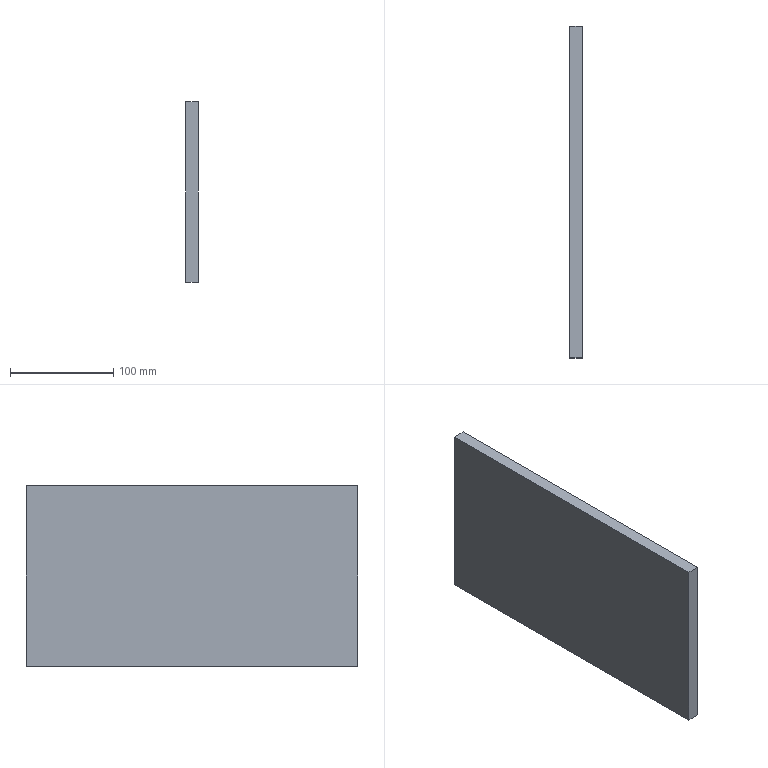Component | NX | CH3404_5-12 | 1 solid | 6 faces | box 12 x 321 x 175 mm | volume 674100 mm3 | plane 6
STEP:
#1=CARTESIAN_POINT('',(0.,0.,0.));
#2=DIRECTION('',(0.,0.,1.));
#3=DIRECTION('',(1.,0.,0.));
#4=AXIS2_PLACEMENT_3D('',#1,#2,#3);
#5=CARTESIAN_POINT('',(-155.,-160.5,1775.));
#6=VERTEX_POINT('',#5);
#7=CARTESIAN_POINT('',(-155.,-160.5,1600.));
#8=VERTEX_POINT('',#7);
#9=CARTESIAN_POINT('',(-155.,-160.5,1775.));
#10=DIRECTION('',(0.,0.,-1.));
#11=VECTOR('',#10,1.);
#12=LINE('',#9,#11);
#13=CARTESIAN_POINT('',(-143.,-160.5,1775.));
#14=DIRECTION('',(0.,1.,0.));
#15=DIRECTION('',(0.,0.,1.));
#16=AXIS2_PLACEMENT_3D('',#13,#14,#15);
#17=PLANE('',#16);
#18=CARTESIAN_POINT('',(0.,-12.));
#19=DIRECTION('',(-1.,0.));
#20=VECTOR('',#19,1.);
#21=LINE('',#18,#20);
#22=(GEOMETRIC_REPRESENTATION_CONTEXT(2)PARAMETRIC_REPRESENTATION_CONTEXT()REPRESENTATION_CONTEXT('',''));
#23=DEFINITIONAL_REPRESENTATION('',(#21),#22);
#24=PCURVE('',#17,#23);
#25=CARTESIAN_POINT('',(-155.,0.,1687.5));
#26=DIRECTION('',(1.,0.,0.));
#27=DIRECTION('',(0.,0.,-1.));
#28=AXIS2_PLACEMENT_3D('',#25,#26,#27);
#29=PLANE('',#28);
#30=CARTESIAN_POINT('',(-87.5,-160.5));
#31=DIRECTION('',(1.,0.));
#32=VECTOR('',#31,1.);
#33=LINE('',#30,#32);
#34=(GEOMETRIC_REPRESENTATION_CONTEXT(2)PARAMETRIC_REPRESENTATION_CONTEXT()REPRESENTATION_CONTEXT('',''));
#35=DEFINITIONAL_REPRESENTATION('',(#33),#34);
#36=PCURVE('',#29,#35);
#37=SURFACE_CURVE('',#12,(#24,#36),.PCURVE_S1.);
#38=EDGE_CURVE('',#6,#8,#37,.T.);
#39=ORIENTED_EDGE('',*,*,#38,.T.);
#40=CARTESIAN_POINT('',(-143.,-160.5,1600.));
#41=VERTEX_POINT('',#40);
#42=CARTESIAN_POINT('',(-143.,-160.5,1600.));
#43=DIRECTION('',(-1.,0.,0.));
#44=VECTOR('',#43,1.);
#45=LINE('',#42,#44);
#46=CARTESIAN_POINT('',(-175.,0.));
#47=DIRECTION('',(0.,-1.));
#48=VECTOR('',#47,1.);
#49=LINE('',#46,#48);
#50=(GEOMETRIC_REPRESENTATION_CONTEXT(2)PARAMETRIC_REPRESENTATION_CONTEXT()REPRESENTATION_CONTEXT('',''));
#51=DEFINITIONAL_REPRESENTATION('',(#49),#50);
#52=PCURVE('',#17,#51);
#53=CARTESIAN_POINT('',(-143.,-160.5,1600.));
#54=DIRECTION('',(0.,0.,1.));
#55=DIRECTION('',(1.,0.,0.));
#56=AXIS2_PLACEMENT_3D('',#53,#54,#55);
#57=PLANE('',#56);
#58=CARTESIAN_POINT('',(0.,0.));
#59=DIRECTION('',(-1.,0.));
#60=VECTOR('',#59,1.);
#61=LINE('',#58,#60);
#62=(GEOMETRIC_REPRESENTATION_CONTEXT(2)PARAMETRIC_REPRESENTATION_CONTEXT()REPRESENTATION_CONTEXT('',''));
#63=DEFINITIONAL_REPRESENTATION('',(#61),#62);
#64=PCURVE('',#57,#63);
#65=SURFACE_CURVE('',#45,(#52,#64),.PCURVE_S1.);
#66=EDGE_CURVE('',#41,#8,#65,.T.);
#67=ORIENTED_EDGE('',*,*,#66,.F.);
#68=CARTESIAN_POINT('',(-143.,-160.5,1775.));
#69=VERTEX_POINT('',#68);
#70=CARTESIAN_POINT('',(-143.,-160.5,1775.));
#71=DIRECTION('',(0.,0.,-1.));
#72=VECTOR('',#71,1.);
#73=LINE('',#70,#72);
#74=CARTESIAN_POINT('',(0.,0.));
#75=DIRECTION('',(-1.,0.));
#76=VECTOR('',#75,1.);
#77=LINE('',#74,#76);
#78=(GEOMETRIC_REPRESENTATION_CONTEXT(2)PARAMETRIC_REPRESENTATION_CONTEXT()REPRESENTATION_CONTEXT('',''));
#79=DEFINITIONAL_REPRESENTATION('',(#77),#78);
#80=PCURVE('',#17,#79);
#81=CARTESIAN_POINT('',(-143.,0.,1687.5));
#82=DIRECTION('',(1.,0.,0.));
#83=DIRECTION('',(0.,0.,-1.));
#84=AXIS2_PLACEMENT_3D('',#81,#82,#83);
#85=PLANE('',#84);
#86=CARTESIAN_POINT('',(-87.5,-160.5));
#87=DIRECTION('',(1.,0.));
#88=VECTOR('',#87,1.);
#89=LINE('',#86,#88);
#90=(GEOMETRIC_REPRESENTATION_CONTEXT(2)PARAMETRIC_REPRESENTATION_CONTEXT()REPRESENTATION_CONTEXT('',''));
#91=DEFINITIONAL_REPRESENTATION('',(#89),#90);
#92=PCURVE('',#85,#91);
#93=SURFACE_CURVE('',#73,(#80,#92),.PCURVE_S1.);
#94=EDGE_CURVE('',#69,#41,#93,.T.);
#95=ORIENTED_EDGE('',*,*,#94,.F.);
#96=CARTESIAN_POINT('',(-143.,-160.5,1775.));
#97=DIRECTION('',(-1.,0.,0.));
#98=VECTOR('',#97,1.);
#99=LINE('',#96,#98);
#100=CARTESIAN_POINT('',(0.,0.));
#101=DIRECTION('',(0.,-1.));
#102=VECTOR('',#101,1.);
#103=LINE('',#100,#102);
#104=(GEOMETRIC_REPRESENTATION_CONTEXT(2)PARAMETRIC_REPRESENTATION_CONTEXT()REPRESENTATION_CONTEXT('',''));
#105=DEFINITIONAL_REPRESENTATION('',(#103),#104);
#106=PCURVE('',#17,#105);
#107=CARTESIAN_POINT('',(-143.,160.5,1775.));
#108=DIRECTION('',(0.,0.,-1.));
#109=DIRECTION('',(-1.,0.,0.));
#110=AXIS2_PLACEMENT_3D('',#107,#108,#109);
#111=PLANE('',#110);
#112=CARTESIAN_POINT('',(0.,-321.));
#113=DIRECTION('',(1.,0.));
#114=VECTOR('',#113,1.);
#115=LINE('',#112,#114);
#116=(GEOMETRIC_REPRESENTATION_CONTEXT(2)PARAMETRIC_REPRESENTATION_CONTEXT()REPRESENTATION_CONTEXT('',''));
#117=DEFINITIONAL_REPRESENTATION('',(#115),#116);
#118=PCURVE('',#111,#117);
#119=SURFACE_CURVE('',#99,(#106,#118),.PCURVE_S1.);
#120=EDGE_CURVE('',#69,#6,#119,.T.);
#121=ORIENTED_EDGE('',*,*,#120,.T.);
#122=EDGE_LOOP('',(#39,#67,#95,#121));
#123=FACE_BOUND('',#122,.T.);
#124=ADVANCED_FACE('',(#123),#17,.F.);
#125=CARTESIAN_POINT('',(-155.,160.5,1600.));
#126=VERTEX_POINT('',#125);
#127=CARTESIAN_POINT('',(-155.,-160.5,1600.));
#128=DIRECTION('',(0.,1.,0.));
#129=VECTOR('',#128,1.);
#130=LINE('',#127,#129);
#131=CARTESIAN_POINT('',(-12.,0.));
#132=DIRECTION('',(0.,1.));
#133=VECTOR('',#132,1.);
#134=LINE('',#131,#133);
#135=(GEOMETRIC_REPRESENTATION_CONTEXT(2)PARAMETRIC_REPRESENTATION_CONTEXT()REPRESENTATION_CONTEXT('',''));
#136=DEFINITIONAL_REPRESENTATION('',(#134),#135);
#137=PCURVE('',#57,#136);
#138=CARTESIAN_POINT('',(87.5,-160.5));
#139=DIRECTION('',(0.,1.));
#140=VECTOR('',#139,1.);
#141=LINE('',#138,#140);
#142=(GEOMETRIC_REPRESENTATION_CONTEXT(2)PARAMETRIC_REPRESENTATION_CONTEXT()REPRESENTATION_CONTEXT('',''));
#143=DEFINITIONAL_REPRESENTATION('',(#141),#142);
#144=PCURVE('',#29,#143);
#145=SURFACE_CURVE('',#130,(#137,#144),.PCURVE_S1.);
#146=EDGE_CURVE('',#8,#126,#145,.T.);
#147=ORIENTED_EDGE('',*,*,#146,.T.);
#148=CARTESIAN_POINT('',(-143.,160.5,1600.));
#149=VERTEX_POINT('',#148);
#150=CARTESIAN_POINT('',(-143.,160.5,1600.));
#151=DIRECTION('',(-1.,0.,0.));
#152=VECTOR('',#151,1.);
#153=LINE('',#150,#152);
#154=CARTESIAN_POINT('',(0.,321.));
#155=DIRECTION('',(-1.,0.));
#156=VECTOR('',#155,1.);
#157=LINE('',#154,#156);
#158=(GEOMETRIC_REPRESENTATION_CONTEXT(2)PARAMETRIC_REPRESENTATION_CONTEXT()REPRESENTATION_CONTEXT('',''));
#159=DEFINITIONAL_REPRESENTATION('',(#157),#158);
#160=PCURVE('',#57,#159);
#161=CARTESIAN_POINT('',(-143.,160.5,1600.));
#162=DIRECTION('',(0.,-1.,0.));
#163=DIRECTION('',(0.,0.,-1.));
#164=AXIS2_PLACEMENT_3D('',#161,#162,#163);
#165=PLANE('',#164);
#166=CARTESIAN_POINT('',(0.,0.));
#167=DIRECTION('',(0.,-1.));
#168=VECTOR('',#167,1.);
#169=LINE('',#166,#168);
#170=(GEOMETRIC_REPRESENTATION_CONTEXT(2)PARAMETRIC_REPRESENTATION_CONTEXT()REPRESENTATION_CONTEXT('',''));
#171=DEFINITIONAL_REPRESENTATION('',(#169),#170);
#172=PCURVE('',#165,#171);
#173=SURFACE_CURVE('',#153,(#160,#172),.PCURVE_S1.);
#174=EDGE_CURVE('',#149,#126,#173,.T.);
#175=ORIENTED_EDGE('',*,*,#174,.F.);
#176=CARTESIAN_POINT('',(-143.,-160.5,1600.));
#177=DIRECTION('',(0.,1.,0.));
#178=VECTOR('',#177,1.);
#179=LINE('',#176,#178);
#180=CARTESIAN_POINT('',(0.,0.));
#181=DIRECTION('',(0.,1.));
#182=VECTOR('',#181,1.);
#183=LINE('',#180,#182);
#184=(GEOMETRIC_REPRESENTATION_CONTEXT(2)PARAMETRIC_REPRESENTATION_CONTEXT()REPRESENTATION_CONTEXT('',''));
#185=DEFINITIONAL_REPRESENTATION('',(#183),#184);
#186=PCURVE('',#57,#185);
#187=CARTESIAN_POINT('',(87.5,-160.5));
#188=DIRECTION('',(0.,1.));
#189=VECTOR('',#188,1.);
#190=LINE('',#187,#189);
#191=(GEOMETRIC_REPRESENTATION_CONTEXT(2)PARAMETRIC_REPRESENTATION_CONTEXT()REPRESENTATION_CONTEXT('',''));
#192=DEFINITIONAL_REPRESENTATION('',(#190),#191);
#193=PCURVE('',#85,#192);
#194=SURFACE_CURVE('',#179,(#186,#193),.PCURVE_S1.);
#195=EDGE_CURVE('',#41,#149,#194,.T.);
#196=ORIENTED_EDGE('',*,*,#195,.F.);
#197=ORIENTED_EDGE('',*,*,#66,.T.);
#198=EDGE_LOOP('',(#147,#175,#196,#197));
#199=FACE_BOUND('',#198,.T.);
#200=ADVANCED_FACE('',(#199),#57,.F.);
#201=CARTESIAN_POINT('',(-155.,160.5,1775.));
#202=VERTEX_POINT('',#201);
#203=CARTESIAN_POINT('',(-155.,160.5,1600.));
#204=DIRECTION('',(0.,0.,1.));
#205=VECTOR('',#204,1.);
#206=LINE('',#203,#205);
#207=CARTESIAN_POINT('',(0.,-12.));
#208=DIRECTION('',(-1.,0.));
#209=VECTOR('',#208,1.);
#210=LINE('',#207,#209);
#211=(GEOMETRIC_REPRESENTATION_CONTEXT(2)PARAMETRIC_REPRESENTATION_CONTEXT()REPRESENTATION_CONTEXT('',''));
#212=DEFINITIONAL_REPRESENTATION('',(#210),#211);
#213=PCURVE('',#165,#212);
#214=CARTESIAN_POINT('',(87.5,160.5));
#215=DIRECTION('',(-1.,0.));
#216=VECTOR('',#215,1.);
#217=LINE('',#214,#216);
#218=(GEOMETRIC_REPRESENTATION_CONTEXT(2)PARAMETRIC_REPRESENTATION_CONTEXT()REPRESENTATION_CONTEXT('',''));
#219=DEFINITIONAL_REPRESENTATION('',(#217),#218);
#220=PCURVE('',#29,#219);
#221=SURFACE_CURVE('',#206,(#213,#220),.PCURVE_S1.);
#222=EDGE_CURVE('',#126,#202,#221,.T.);
#223=ORIENTED_EDGE('',*,*,#222,.T.);
#224=CARTESIAN_POINT('',(-143.,160.5,1775.));
#225=VERTEX_POINT('',#224);
#226=CARTESIAN_POINT('',(-143.,160.5,1775.));
#227=DIRECTION('',(-1.,0.,0.));
#228=VECTOR('',#227,1.);
#229=LINE('',#226,#228);
#230=CARTESIAN_POINT('',(-175.,0.));
#231=DIRECTION('',(0.,-1.));
#232=VECTOR('',#231,1.);
#233=LINE('',#230,#232);
#234=(GEOMETRIC_REPRESENTATION_CONTEXT(2)PARAMETRIC_REPRESENTATION_CONTEXT()REPRESENTATION_CONTEXT('',''));
#235=DEFINITIONAL_REPRESENTATION('',(#233),#234);
#236=PCURVE('',#165,#235);
#237=CARTESIAN_POINT('',(0.,0.));
#238=DIRECTION('',(1.,0.));
#239=VECTOR('',#238,1.);
#240=LINE('',#237,#239);
#241=(GEOMETRIC_REPRESENTATION_CONTEXT(2)PARAMETRIC_REPRESENTATION_CONTEXT()REPRESENTATION_CONTEXT('',''));
#242=DEFINITIONAL_REPRESENTATION('',(#240),#241);
#243=PCURVE('',#111,#242);
#244=SURFACE_CURVE('',#229,(#236,#243),.PCURVE_S1.);
#245=EDGE_CURVE('',#225,#202,#244,.T.);
#246=ORIENTED_EDGE('',*,*,#245,.F.);
#247=CARTESIAN_POINT('',(-143.,160.5,1600.));
#248=DIRECTION('',(0.,0.,1.));
#249=VECTOR('',#248,1.);
#250=LINE('',#247,#249);
#251=CARTESIAN_POINT('',(0.,0.));
#252=DIRECTION('',(-1.,0.));
#253=VECTOR('',#252,1.);
#254=LINE('',#251,#253);
#255=(GEOMETRIC_REPRESENTATION_CONTEXT(2)PARAMETRIC_REPRESENTATION_CONTEXT()REPRESENTATION_CONTEXT('',''));
#256=DEFINITIONAL_REPRESENTATION('',(#254),#255);
#257=PCURVE('',#165,#256);
#258=CARTESIAN_POINT('',(87.5,160.5));
#259=DIRECTION('',(-1.,0.));
#260=VECTOR('',#259,1.);
#261=LINE('',#258,#260);
#262=(GEOMETRIC_REPRESENTATION_CONTEXT(2)PARAMETRIC_REPRESENTATION_CONTEXT()REPRESENTATION_CONTEXT('',''));
#263=DEFINITIONAL_REPRESENTATION('',(#261),#262);
#264=PCURVE('',#85,#263);
#265=SURFACE_CURVE('',#250,(#257,#264),.PCURVE_S1.);
#266=EDGE_CURVE('',#149,#225,#265,.T.);
#267=ORIENTED_EDGE('',*,*,#266,.F.);
#268=ORIENTED_EDGE('',*,*,#174,.T.);
#269=EDGE_LOOP('',(#223,#246,#267,#268));
#270=FACE_BOUND('',#269,.T.);
#271=ADVANCED_FACE('',(#270),#165,.F.);
#272=CARTESIAN_POINT('',(-155.,160.5,1775.));
#273=DIRECTION('',(0.,-1.,0.));
#274=VECTOR('',#273,1.);
#275=LINE('',#272,#274);
#276=CARTESIAN_POINT('',(12.,0.));
#277=DIRECTION('',(0.,-1.));
#278=VECTOR('',#277,1.);
#279=LINE('',#276,#278);
#280=(GEOMETRIC_REPRESENTATION_CONTEXT(2)PARAMETRIC_REPRESENTATION_CONTEXT()REPRESENTATION_CONTEXT('',''));
#281=DEFINITIONAL_REPRESENTATION('',(#279),#280);
#282=PCURVE('',#111,#281);
#283=CARTESIAN_POINT('',(-87.5,160.5));
#284=DIRECTION('',(0.,-1.));
#285=VECTOR('',#284,1.);
#286=LINE('',#283,#285);
#287=(GEOMETRIC_REPRESENTATION_CONTEXT(2)PARAMETRIC_REPRESENTATION_CONTEXT()REPRESENTATION_CONTEXT('',''));
#288=DEFINITIONAL_REPRESENTATION('',(#286),#287);
#289=PCURVE('',#29,#288);
#290=SURFACE_CURVE('',#275,(#282,#289),.PCURVE_S1.);
#291=EDGE_CURVE('',#202,#6,#290,.T.);
#292=ORIENTED_EDGE('',*,*,#291,.T.);
#293=ORIENTED_EDGE('',*,*,#120,.F.);
#294=CARTESIAN_POINT('',(-143.,160.5,1775.));
#295=DIRECTION('',(0.,-1.,0.));
#296=VECTOR('',#295,1.);
#297=LINE('',#294,#296);
#298=CARTESIAN_POINT('',(0.,0.));
#299=DIRECTION('',(0.,-1.));
#300=VECTOR('',#299,1.);
#301=LINE('',#298,#300);
#302=(GEOMETRIC_REPRESENTATION_CONTEXT(2)PARAMETRIC_REPRESENTATION_CONTEXT()REPRESENTATION_CONTEXT('',''));
#303=DEFINITIONAL_REPRESENTATION('',(#301),#302);
#304=PCURVE('',#111,#303);
#305=CARTESIAN_POINT('',(-87.5,160.5));
#306=DIRECTION('',(0.,-1.));
#307=VECTOR('',#306,1.);
#308=LINE('',#305,#307);
#309=(GEOMETRIC_REPRESENTATION_CONTEXT(2)PARAMETRIC_REPRESENTATION_CONTEXT()REPRESENTATION_CONTEXT('',''));
#310=DEFINITIONAL_REPRESENTATION('',(#308),#309);
#311=PCURVE('',#85,#310);
#312=SURFACE_CURVE('',#297,(#304,#311),.PCURVE_S1.);
#313=EDGE_CURVE('',#225,#69,#312,.T.);
#314=ORIENTED_EDGE('',*,*,#313,.F.);
#315=ORIENTED_EDGE('',*,*,#245,.T.);
#316=EDGE_LOOP('',(#292,#293,#314,#315));
#317=FACE_BOUND('',#316,.T.);
#318=ADVANCED_FACE('',(#317),#111,.F.);
#319=ORIENTED_EDGE('',*,*,#94,.T.);
#320=ORIENTED_EDGE('',*,*,#195,.T.);
#321=ORIENTED_EDGE('',*,*,#266,.T.);
#322=ORIENTED_EDGE('',*,*,#313,.T.);
#323=EDGE_LOOP('',(#319,#320,#321,#322));
#324=FACE_BOUND('',#323,.T.);
#325=ADVANCED_FACE('',(#324),#85,.T.);
#326=ORIENTED_EDGE('',*,*,#38,.F.);
#327=ORIENTED_EDGE('',*,*,#291,.F.);
#328=ORIENTED_EDGE('',*,*,#222,.F.);
#329=ORIENTED_EDGE('',*,*,#146,.F.);
#330=EDGE_LOOP('',(#326,#327,#328,#329));
#331=FACE_BOUND('',#330,.T.);
#332=ADVANCED_FACE('',(#331),#29,.F.);
#333=CLOSED_SHELL('',(#124,#200,#271,#318,#325,#332));
#334=MANIFOLD_SOLID_BREP('',#333);
#335=(LENGTH_UNIT()NAMED_UNIT(*)SI_UNIT(.MILLI.,.METRE.));
#336=UNCERTAINTY_MEASURE_WITH_UNIT(LENGTH_MEASURE(0.0000001),#335,'','');
#337=(NAMED_UNIT(*)PLANE_ANGLE_UNIT()SI_UNIT($,.RADIAN.));
#338=(NAMED_UNIT(*)SI_UNIT($,.STERADIAN.)SOLID_ANGLE_UNIT());
#339=(GEOMETRIC_REPRESENTATION_CONTEXT(3)GLOBAL_UNCERTAINTY_ASSIGNED_CONTEXT((#336))GLOBAL_UNIT_ASSIGNED_CONTEXT((#335,#337,#338))REPRESENTATION_CONTEXT('',''));
#340=ADVANCED_BREP_SHAPE_REPRESENTATION('',(#4,#334),#339);